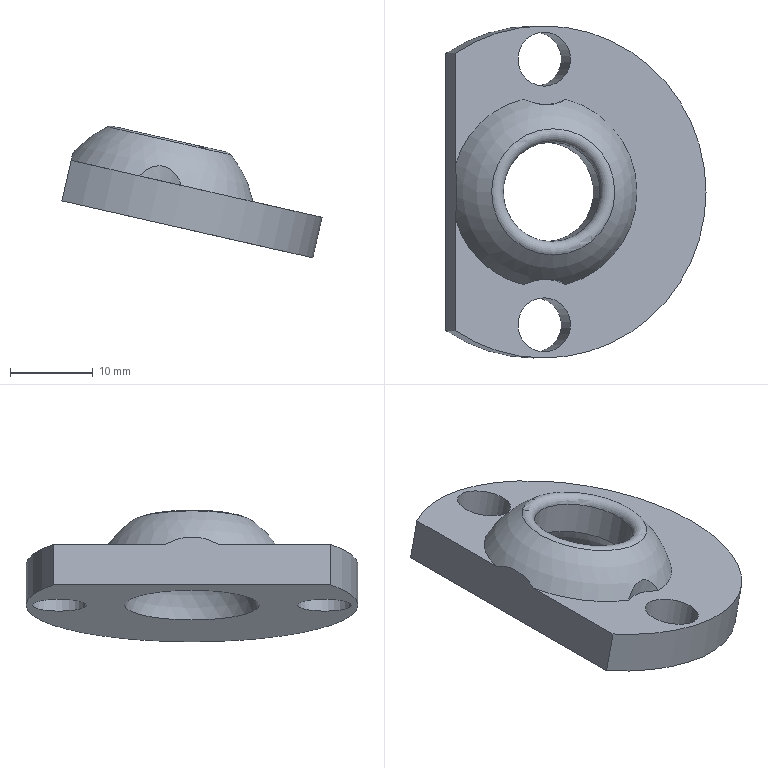Component | NX | COVER | 1 solid | 12 faces | volume 4955 mm3 | cylinder 6 | plane 3 | sphere 2 | torus 1 | commonest cylinder face diameters 11 x2 6.5 x2 40 x1 12 x1